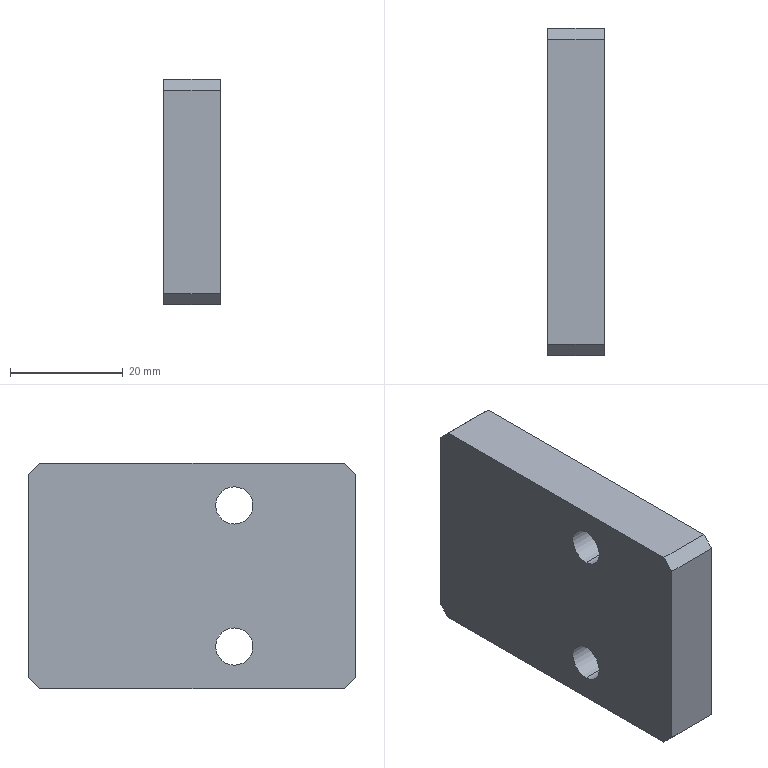Component | SolidWorks | NewDieSet-1_MoldSlotBaffle-7 | 1 solid | 14 faces | box 10 x 58 x 40 mm | volume 22436 mm3 | plane 10 | cylinder 4 | commonest cylinder face diameters 6.6 x4
build123d program:
from build123d import *

# Parameters (mm, degrees)
SKETCH1_W                = 58
SKETCH1_H                = 40
BOSS_EXTRUDE1_DEPTH      = 10
CHAMFER1_SIZE            = 2
M6_CLEARANCE_HOLE1_D     = 6.6
M6_CLEARANCE_HOLE1_DEPTH = 25.2
M6_CLEARANCE_HOLE1_TIP   = 1.983


with BuildPart() as part:
    # Sketch1 → Boss-Extrude1 (new body)
    with BuildSketch(Plane(origin=(0, 0, 0), x_dir=(1, 0, 0), z_dir=(0, 1, 0))):
        with Locations((29, 20)):
            Rectangle(SKETCH1_W, SKETCH1_H)
    extrude(amount=BOSS_EXTRUDE1_DEPTH)

    # Chamfer1
    chamfer1_edges = [part.edges().sort_by_distance(p)[0] for p in [
        (0, 5, -40),
        (58, 5, -40),
        (58, 5, 0),
        (0, 5, 0),
    ]]
    chamfer(chamfer1_edges, length=CHAMFER1_SIZE)

    # M6 Clearance Hole1
    with Locations(Plane(origin=(0, 10, 0), x_dir=(1, 0, 0), z_dir=(0, 1, 0))):
        with Locations((36.5, 7.5), (36.5, 32.5)):
            Hole(M6_CLEARANCE_HOLE1_D / 2, depth=M6_CLEARANCE_HOLE1_DEPTH)
            with Locations((0, 0, -(M6_CLEARANCE_HOLE1_DEPTH + M6_CLEARANCE_HOLE1_TIP / 2))):  # 118° drill point
                Cone(0, M6_CLEARANCE_HOLE1_D / 2, M6_CLEARANCE_HOLE1_TIP, mode=Mode.SUBTRACT)


solid = part.part

# Placed as in the assembly
solid = solid.moved(Location((143.254, 22.427, 215.5), (0, 0, -90)))
STEP:
#1=COLOUR_RGB('',0.7922,0.8196,0.9333);
#2=FILL_AREA_STYLE_COLOUR('',#1);
#3=FILL_AREA_STYLE('',(#2));
#4=SURFACE_STYLE_FILL_AREA(#3);
#5=SURFACE_SIDE_STYLE('',(#4));
#6=SURFACE_STYLE_USAGE(.BOTH.,#5);
#7=PRESENTATION_STYLE_ASSIGNMENT((#6));
#8=CARTESIAN_POINT('',(5.64,-0.5541,8.319));
#9=VERTEX_POINT('',#8);
#10=CARTESIAN_POINT('',(5.64,-0.5541,8.059));
#11=VERTEX_POINT('',#10);
#12=CARTESIAN_POINT('',(5.64,-0.5541,8.189));
#13=DIRECTION('',(-1.,0.,-0.));
#14=DIRECTION('',(0.,0.,-1.));
#15=AXIS2_PLACEMENT_3D('',#12,#13,#14);
#16=CIRCLE('',#15,0.1299);
#17=EDGE_CURVE('',#9,#11,#16,.T.);
#18=ORIENTED_EDGE('',*,*,#17,.T.);
#19=CARTESIAN_POINT('',(6.034,-0.5541,8.059));
#20=VERTEX_POINT('',#19);
#21=CARTESIAN_POINT('',(6.034,-0.5541,8.059));
#22=DIRECTION('',(1.,-0.,0.));
#23=VECTOR('',#22,39.37);
#24=LINE('',#21,#23);
#25=EDGE_CURVE('',#11,#20,#24,.T.);
#26=ORIENTED_EDGE('',*,*,#25,.T.);
#27=CARTESIAN_POINT('',(6.034,-0.5541,8.319));
#28=VERTEX_POINT('',#27);
#29=CARTESIAN_POINT('',(6.034,-0.5541,8.189));
#30=DIRECTION('',(1.,-0.,0.));
#31=DIRECTION('',(0.,0.,1.));
#32=AXIS2_PLACEMENT_3D('',#29,#30,#31);
#33=CIRCLE('',#32,0.1299);
#34=EDGE_CURVE('',#20,#28,#33,.T.);
#35=ORIENTED_EDGE('',*,*,#34,.T.);
#36=CARTESIAN_POINT('',(6.034,-0.5541,8.319));
#37=DIRECTION('',(1.,-0.,0.));
#38=VECTOR('',#37,39.37);
#39=LINE('',#36,#38);
#40=EDGE_CURVE('',#9,#28,#39,.T.);
#41=ORIENTED_EDGE('',*,*,#40,.F.);
#42=EDGE_LOOP('',(#18,#26,#35,#41));
#43=FACE_OUTER_BOUND('',#42,.T.);
#44=CARTESIAN_POINT('',(6.034,-0.5541,8.189));
#45=DIRECTION('',(1.,-0.,0.));
#46=DIRECTION('',(0.,0.,1.));
#47=AXIS2_PLACEMENT_3D('',#44,#45,#46);
#48=CYLINDRICAL_SURFACE('',#47,0.1299);
#49=ADVANCED_FACE('',(#43),#48,.F.);
#50=CARTESIAN_POINT('',(5.64,-0.5541,7.335));
#51=VERTEX_POINT('',#50);
#52=CARTESIAN_POINT('',(5.64,-0.5541,7.075));
#53=VERTEX_POINT('',#52);
#54=CARTESIAN_POINT('',(5.64,-0.5541,7.205));
#55=DIRECTION('',(-1.,0.,-0.));
#56=DIRECTION('',(0.,0.,-1.));
#57=AXIS2_PLACEMENT_3D('',#54,#55,#56);
#58=CIRCLE('',#57,0.1299);
#59=EDGE_CURVE('',#51,#53,#58,.T.);
#60=ORIENTED_EDGE('',*,*,#59,.T.);
#61=CARTESIAN_POINT('',(6.034,-0.5541,7.075));
#62=VERTEX_POINT('',#61);
#63=CARTESIAN_POINT('',(6.034,-0.5541,7.075));
#64=DIRECTION('',(1.,-0.,0.));
#65=VECTOR('',#64,39.37);
#66=LINE('',#63,#65);
#67=EDGE_CURVE('',#53,#62,#66,.T.);
#68=ORIENTED_EDGE('',*,*,#67,.T.);
#69=CARTESIAN_POINT('',(6.034,-0.5541,7.335));
#70=VERTEX_POINT('',#69);
#71=CARTESIAN_POINT('',(6.034,-0.5541,7.205));
#72=DIRECTION('',(1.,-0.,0.));
#73=DIRECTION('',(0.,0.,1.));
#74=AXIS2_PLACEMENT_3D('',#71,#72,#73);
#75=CIRCLE('',#74,0.1299);
#76=EDGE_CURVE('',#62,#70,#75,.T.);
#77=ORIENTED_EDGE('',*,*,#76,.T.);
#78=CARTESIAN_POINT('',(6.034,-0.5541,7.335));
#79=DIRECTION('',(1.,-0.,0.));
#80=VECTOR('',#79,39.37);
#81=LINE('',#78,#80);
#82=EDGE_CURVE('',#51,#70,#81,.T.);
#83=ORIENTED_EDGE('',*,*,#82,.F.);
#84=EDGE_LOOP('',(#60,#68,#77,#83));
#85=FACE_OUTER_BOUND('',#84,.T.);
#86=CARTESIAN_POINT('',(6.034,-0.5541,7.205));
#87=DIRECTION('',(1.,-0.,0.));
#88=DIRECTION('',(0.,0.,1.));
#89=AXIS2_PLACEMENT_3D('',#86,#87,#88);
#90=CYLINDRICAL_SURFACE('',#89,0.1299);
#91=ADVANCED_FACE('',(#85),#90,.F.);
#92=CARTESIAN_POINT('',(5.64,0.883,6.988));
#93=VERTEX_POINT('',#92);
#94=CARTESIAN_POINT('',(5.64,0.883,8.406));
#95=VERTEX_POINT('',#94);
#96=CARTESIAN_POINT('',(5.64,0.883,8.484));
#97=DIRECTION('',(-0.,0.,1.));
#98=VECTOR('',#97,39.37);
#99=LINE('',#96,#98);
#100=EDGE_CURVE('',#93,#95,#99,.T.);
#101=ORIENTED_EDGE('',*,*,#100,.T.);
#102=CARTESIAN_POINT('',(6.034,0.883,8.406));
#103=VERTEX_POINT('',#102);
#104=CARTESIAN_POINT('',(6.034,0.883,8.406));
#105=DIRECTION('',(1.,-0.,0.));
#106=VECTOR('',#105,39.37);
#107=LINE('',#104,#106);
#108=EDGE_CURVE('',#95,#103,#107,.T.);
#109=ORIENTED_EDGE('',*,*,#108,.T.);
#110=CARTESIAN_POINT('',(6.034,0.883,6.988));
#111=VERTEX_POINT('',#110);
#112=CARTESIAN_POINT('',(6.034,0.883,8.484));
#113=DIRECTION('',(-0.,0.,1.));
#114=VECTOR('',#113,39.37);
#115=LINE('',#112,#114);
#116=EDGE_CURVE('',#111,#103,#115,.T.);
#117=ORIENTED_EDGE('',*,*,#116,.F.);
#118=CARTESIAN_POINT('',(6.034,0.883,6.988));
#119=DIRECTION('',(-1.,0.,-0.));
#120=VECTOR('',#119,39.37);
#121=LINE('',#118,#120);
#122=EDGE_CURVE('',#111,#93,#121,.T.);
#123=ORIENTED_EDGE('',*,*,#122,.T.);
#124=EDGE_LOOP('',(#101,#109,#117,#123));
#125=FACE_OUTER_BOUND('',#124,.T.);
#126=CARTESIAN_POINT('',(6.034,0.883,8.484));
#127=DIRECTION('',(-0.,-1.,0.));
#128=DIRECTION('',(0.,-0.,-1.));
#129=AXIS2_PLACEMENT_3D('',#126,#127,#128);
#130=PLANE('',#129);
#131=ADVANCED_FACE('',(#125),#130,.F.);
#132=CARTESIAN_POINT('',(6.034,0.8042,8.484));
#133=VERTEX_POINT('',#132);
#134=CARTESIAN_POINT('',(6.034,-1.322,8.484));
#135=VERTEX_POINT('',#134);
#136=CARTESIAN_POINT('',(6.034,0.883,8.484));
#137=DIRECTION('',(-0.,-1.,0.));
#138=VECTOR('',#137,39.37);
#139=LINE('',#136,#138);
#140=EDGE_CURVE('',#133,#135,#139,.T.);
#141=ORIENTED_EDGE('',*,*,#140,.F.);
#142=CARTESIAN_POINT('',(5.64,0.8042,8.484));
#143=VERTEX_POINT('',#142);
#144=CARTESIAN_POINT('',(6.034,0.8042,8.484));
#145=DIRECTION('',(-1.,0.,-0.));
#146=VECTOR('',#145,39.37);
#147=LINE('',#144,#146);
#148=EDGE_CURVE('',#133,#143,#147,.T.);
#149=ORIENTED_EDGE('',*,*,#148,.T.);
#150=CARTESIAN_POINT('',(5.64,-1.322,8.484));
#151=VERTEX_POINT('',#150);
#152=CARTESIAN_POINT('',(5.64,0.883,8.484));
#153=DIRECTION('',(-0.,-1.,0.));
#154=VECTOR('',#153,39.37);
#155=LINE('',#152,#154);
#156=EDGE_CURVE('',#143,#151,#155,.T.);
#157=ORIENTED_EDGE('',*,*,#156,.T.);
#158=CARTESIAN_POINT('',(6.034,-1.322,8.484));
#159=DIRECTION('',(1.,-0.,0.));
#160=VECTOR('',#159,39.37);
#161=LINE('',#158,#160);
#162=EDGE_CURVE('',#151,#135,#161,.T.);
#163=ORIENTED_EDGE('',*,*,#162,.T.);
#164=EDGE_LOOP('',(#141,#149,#157,#163));
#165=FACE_OUTER_BOUND('',#164,.T.);
#166=CARTESIAN_POINT('',(6.034,0.883,8.484));
#167=DIRECTION('',(0.,-0.,-1.));
#168=DIRECTION('',(0.,1.,-0.));
#169=AXIS2_PLACEMENT_3D('',#166,#167,#168);
#170=PLANE('',#169);
#171=ADVANCED_FACE('',(#165),#170,.F.);
#172=CARTESIAN_POINT('',(6.034,-1.401,8.406));
#173=VERTEX_POINT('',#172);
#174=CARTESIAN_POINT('',(6.034,-1.401,6.988));
#175=VERTEX_POINT('',#174);
#176=CARTESIAN_POINT('',(6.034,-1.401,8.484));
#177=DIRECTION('',(0.,-0.,-1.));
#178=VECTOR('',#177,39.37);
#179=LINE('',#176,#178);
#180=EDGE_CURVE('',#173,#175,#179,.T.);
#181=ORIENTED_EDGE('',*,*,#180,.F.);
#182=CARTESIAN_POINT('',(5.64,-1.401,8.406));
#183=VERTEX_POINT('',#182);
#184=CARTESIAN_POINT('',(6.034,-1.401,8.406));
#185=DIRECTION('',(-1.,0.,-0.));
#186=VECTOR('',#185,39.37);
#187=LINE('',#184,#186);
#188=EDGE_CURVE('',#173,#183,#187,.T.);
#189=ORIENTED_EDGE('',*,*,#188,.T.);
#190=CARTESIAN_POINT('',(5.64,-1.401,6.988));
#191=VERTEX_POINT('',#190);
#192=CARTESIAN_POINT('',(5.64,-1.401,8.484));
#193=DIRECTION('',(0.,-0.,-1.));
#194=VECTOR('',#193,39.37);
#195=LINE('',#192,#194);
#196=EDGE_CURVE('',#183,#191,#195,.T.);
#197=ORIENTED_EDGE('',*,*,#196,.T.);
#198=CARTESIAN_POINT('',(6.034,-1.401,6.988));
#199=DIRECTION('',(1.,-0.,0.));
#200=VECTOR('',#199,39.37);
#201=LINE('',#198,#200);
#202=EDGE_CURVE('',#191,#175,#201,.T.);
#203=ORIENTED_EDGE('',*,*,#202,.T.);
#204=EDGE_LOOP('',(#181,#189,#197,#203));
#205=FACE_OUTER_BOUND('',#204,.T.);
#206=CARTESIAN_POINT('',(6.034,-1.401,8.484));
#207=DIRECTION('',(0.,1.,-0.));
#208=DIRECTION('',(-0.,0.,1.));
#209=AXIS2_PLACEMENT_3D('',#206,#207,#208);
#210=PLANE('',#209);
#211=ADVANCED_FACE('',(#205),#210,.F.);
#212=CARTESIAN_POINT('',(6.034,-1.322,6.909));
#213=VERTEX_POINT('',#212);
#214=CARTESIAN_POINT('',(6.034,0.8042,6.909));
#215=VERTEX_POINT('',#214);
#216=CARTESIAN_POINT('',(6.034,0.883,6.909));
#217=DIRECTION('',(0.,1.,-0.));
#218=VECTOR('',#217,39.37);
#219=LINE('',#216,#218);
#220=EDGE_CURVE('',#213,#215,#219,.T.);
#221=ORIENTED_EDGE('',*,*,#220,.F.);
#222=CARTESIAN_POINT('',(5.64,-1.322,6.909));
#223=VERTEX_POINT('',#222);
#224=CARTESIAN_POINT('',(6.034,-1.322,6.909));
#225=DIRECTION('',(-1.,0.,-0.));
#226=VECTOR('',#225,39.37);
#227=LINE('',#224,#226);
#228=EDGE_CURVE('',#213,#223,#227,.T.);
#229=ORIENTED_EDGE('',*,*,#228,.T.);
#230=CARTESIAN_POINT('',(5.64,0.8042,6.909));
#231=VERTEX_POINT('',#230);
#232=CARTESIAN_POINT('',(5.64,0.883,6.909));
#233=DIRECTION('',(0.,1.,-0.));
#234=VECTOR('',#233,39.37);
#235=LINE('',#232,#234);
#236=EDGE_CURVE('',#223,#231,#235,.T.);
#237=ORIENTED_EDGE('',*,*,#236,.T.);
#238=CARTESIAN_POINT('',(6.034,0.8042,6.909));
#239=DIRECTION('',(1.,-0.,0.));
#240=VECTOR('',#239,39.37);
#241=LINE('',#238,#240);
#242=EDGE_CURVE('',#231,#215,#241,.T.);
#243=ORIENTED_EDGE('',*,*,#242,.T.);
#244=EDGE_LOOP('',(#221,#229,#237,#243));
#245=FACE_OUTER_BOUND('',#244,.T.);
#246=CARTESIAN_POINT('',(6.034,0.883,6.909));
#247=DIRECTION('',(-0.,0.,1.));
#248=DIRECTION('',(-0.,-1.,0.));
#249=AXIS2_PLACEMENT_3D('',#246,#247,#248);
#250=PLANE('',#249);
#251=ADVANCED_FACE('',(#245),#250,.F.);
#252=CARTESIAN_POINT('',(6.034,-0.5541,8.189));
#253=DIRECTION('',(1.,-0.,0.));
#254=DIRECTION('',(0.,0.,1.));
#255=AXIS2_PLACEMENT_3D('',#252,#253,#254);
#256=CIRCLE('',#255,0.1299);
#257=EDGE_CURVE('',#28,#20,#256,.T.);
#258=ORIENTED_EDGE('',*,*,#257,.F.);
#259=ORIENTED_EDGE('',*,*,#34,.F.);
#260=EDGE_LOOP('',(#258,#259));
#261=FACE_BOUND('',#260,.T.);
#262=CARTESIAN_POINT('',(6.034,-0.5541,7.205));
#263=DIRECTION('',(1.,-0.,0.));
#264=DIRECTION('',(0.,0.,1.));
#265=AXIS2_PLACEMENT_3D('',#262,#263,#264);
#266=CIRCLE('',#265,0.1299);
#267=EDGE_CURVE('',#70,#62,#266,.T.);
#268=ORIENTED_EDGE('',*,*,#267,.F.);
#269=ORIENTED_EDGE('',*,*,#76,.F.);
#270=EDGE_LOOP('',(#268,#269));
#271=FACE_BOUND('',#270,.T.);
#272=ORIENTED_EDGE('',*,*,#116,.T.);
#273=CARTESIAN_POINT('',(6.034,0.8042,8.484));
#274=DIRECTION('',(-0.,-0.7071,0.7071));
#275=VECTOR('',#274,39.37);
#276=LINE('',#273,#275);
#277=EDGE_CURVE('',#103,#133,#276,.T.);
#278=ORIENTED_EDGE('',*,*,#277,.T.);
#279=ORIENTED_EDGE('',*,*,#140,.T.);
#280=CARTESIAN_POINT('',(6.034,-1.401,8.406));
#281=DIRECTION('',(0.,-0.7071,-0.7071));
#282=VECTOR('',#281,39.37);
#283=LINE('',#280,#282);
#284=EDGE_CURVE('',#135,#173,#283,.T.);
#285=ORIENTED_EDGE('',*,*,#284,.T.);
#286=ORIENTED_EDGE('',*,*,#180,.T.);
#287=CARTESIAN_POINT('',(6.034,-1.322,6.909));
#288=DIRECTION('',(0.,0.7071,-0.7071));
#289=VECTOR('',#288,39.37);
#290=LINE('',#287,#289);
#291=EDGE_CURVE('',#175,#213,#290,.T.);
#292=ORIENTED_EDGE('',*,*,#291,.T.);
#293=ORIENTED_EDGE('',*,*,#220,.T.);
#294=CARTESIAN_POINT('',(6.034,0.883,6.988));
#295=DIRECTION('',(-0.,0.7071,0.7071));
#296=VECTOR('',#295,39.37);
#297=LINE('',#294,#296);
#298=EDGE_CURVE('',#215,#111,#297,.T.);
#299=ORIENTED_EDGE('',*,*,#298,.T.);
#300=EDGE_LOOP('',(#272,#278,#279,#285,#286,#292,#293,#299));
#301=FACE_OUTER_BOUND('',#300,.T.);
#302=CARTESIAN_POINT('',(6.034,0.883,8.484));
#303=DIRECTION('',(-1.,0.,-0.));
#304=DIRECTION('',(0.,-0.,-1.));
#305=AXIS2_PLACEMENT_3D('',#302,#303,#304);
#306=PLANE('',#305);
#307=ADVANCED_FACE('',(#261,#271,#301),#306,.F.);
#308=ORIENTED_EDGE('',*,*,#17,.F.);
#309=CARTESIAN_POINT('',(5.64,-0.5541,8.189));
#310=DIRECTION('',(-1.,0.,-0.));
#311=DIRECTION('',(0.,0.,-1.));
#312=AXIS2_PLACEMENT_3D('',#309,#310,#311);
#313=CIRCLE('',#312,0.1299);
#314=EDGE_CURVE('',#11,#9,#313,.T.);
#315=ORIENTED_EDGE('',*,*,#314,.F.);
#316=EDGE_LOOP('',(#308,#315));
#317=FACE_BOUND('',#316,.T.);
#318=ORIENTED_EDGE('',*,*,#59,.F.);
#319=CARTESIAN_POINT('',(5.64,-0.5541,7.205));
#320=DIRECTION('',(-1.,0.,-0.));
#321=DIRECTION('',(0.,0.,-1.));
#322=AXIS2_PLACEMENT_3D('',#319,#320,#321);
#323=CIRCLE('',#322,0.1299);
#324=EDGE_CURVE('',#53,#51,#323,.T.);
#325=ORIENTED_EDGE('',*,*,#324,.F.);
#326=EDGE_LOOP('',(#318,#325));
#327=FACE_BOUND('',#326,.T.);
#328=ORIENTED_EDGE('',*,*,#156,.F.);
#329=CARTESIAN_POINT('',(5.64,0.8436,8.445));
#330=DIRECTION('',(0.,0.7071,-0.7071));
#331=VECTOR('',#330,39.37);
#332=LINE('',#329,#331);
#333=EDGE_CURVE('',#143,#95,#332,.T.);
#334=ORIENTED_EDGE('',*,*,#333,.T.);
#335=ORIENTED_EDGE('',*,*,#100,.F.);
#336=CARTESIAN_POINT('',(5.64,1.631,7.736));
#337=DIRECTION('',(0.,-0.7071,-0.7071));
#338=VECTOR('',#337,39.37);
#339=LINE('',#336,#338);
#340=EDGE_CURVE('',#93,#231,#339,.T.);
#341=ORIENTED_EDGE('',*,*,#340,.T.);
#342=ORIENTED_EDGE('',*,*,#236,.F.);
#343=CARTESIAN_POINT('',(5.64,-1.007,6.594));
#344=DIRECTION('',(-0.,-0.7071,0.7071));
#345=VECTOR('',#344,39.37);
#346=LINE('',#343,#345);
#347=EDGE_CURVE('',#223,#191,#346,.T.);
#348=ORIENTED_EDGE('',*,*,#347,.T.);
#349=ORIENTED_EDGE('',*,*,#196,.F.);
#350=CARTESIAN_POINT('',(5.64,-0.2194,9.587));
#351=DIRECTION('',(-0.,0.7071,0.7071));
#352=VECTOR('',#351,39.37);
#353=LINE('',#350,#352);
#354=EDGE_CURVE('',#183,#151,#353,.T.);
#355=ORIENTED_EDGE('',*,*,#354,.T.);
#356=EDGE_LOOP('',(#328,#334,#335,#341,#342,#348,#349,#355));
#357=FACE_OUTER_BOUND('',#356,.T.);
#358=CARTESIAN_POINT('',(5.64,0.883,8.484));
#359=DIRECTION('',(-1.,0.,-0.));
#360=DIRECTION('',(0.,-0.,-1.));
#361=AXIS2_PLACEMENT_3D('',#358,#359,#360);
#362=PLANE('',#361);
#363=ADVANCED_FACE('',(#317,#327,#357),#362,.T.);
#364=ORIENTED_EDGE('',*,*,#277,.F.);
#365=ORIENTED_EDGE('',*,*,#108,.F.);
#366=ORIENTED_EDGE('',*,*,#333,.F.);
#367=ORIENTED_EDGE('',*,*,#148,.F.);
#368=EDGE_LOOP('',(#364,#365,#366,#367));
#369=FACE_OUTER_BOUND('',#368,.T.);
#370=CARTESIAN_POINT('',(6.034,0.8042,8.484));
#371=DIRECTION('',(0.,-0.7071,-0.7071));
#372=DIRECTION('',(-1.,0.,-0.));
#373=AXIS2_PLACEMENT_3D('',#370,#371,#372);
#374=PLANE('',#373);
#375=ADVANCED_FACE('',(#369),#374,.F.);
#376=ORIENTED_EDGE('',*,*,#284,.F.);
#377=ORIENTED_EDGE('',*,*,#162,.F.);
#378=ORIENTED_EDGE('',*,*,#354,.F.);
#379=ORIENTED_EDGE('',*,*,#188,.F.);
#380=EDGE_LOOP('',(#376,#377,#378,#379));
#381=FACE_OUTER_BOUND('',#380,.T.);
#382=CARTESIAN_POINT('',(6.034,-1.401,8.406));
#383=DIRECTION('',(0.,0.7071,-0.7071));
#384=DIRECTION('',(-1.,0.,-0.));
#385=AXIS2_PLACEMENT_3D('',#382,#383,#384);
#386=PLANE('',#385);
#387=ADVANCED_FACE('',(#381),#386,.F.);
#388=ORIENTED_EDGE('',*,*,#291,.F.);
#389=ORIENTED_EDGE('',*,*,#202,.F.);
#390=ORIENTED_EDGE('',*,*,#347,.F.);
#391=ORIENTED_EDGE('',*,*,#228,.F.);
#392=EDGE_LOOP('',(#388,#389,#390,#391));
#393=FACE_OUTER_BOUND('',#392,.T.);
#394=CARTESIAN_POINT('',(6.034,-1.322,6.909));
#395=DIRECTION('',(-0.,0.7071,0.7071));
#396=DIRECTION('',(-1.,0.,-0.));
#397=AXIS2_PLACEMENT_3D('',#394,#395,#396);
#398=PLANE('',#397);
#399=ADVANCED_FACE('',(#393),#398,.F.);
#400=ORIENTED_EDGE('',*,*,#298,.F.);
#401=ORIENTED_EDGE('',*,*,#242,.F.);
#402=ORIENTED_EDGE('',*,*,#340,.F.);
#403=ORIENTED_EDGE('',*,*,#122,.F.);
#404=EDGE_LOOP('',(#400,#401,#402,#403));
#405=FACE_OUTER_BOUND('',#404,.T.);
#406=CARTESIAN_POINT('',(6.034,0.883,6.988));
#407=DIRECTION('',(-0.,-0.7071,0.7071));
#408=DIRECTION('',(-1.,0.,-0.));
#409=AXIS2_PLACEMENT_3D('',#406,#407,#408);
#410=PLANE('',#409);
#411=ADVANCED_FACE('',(#405),#410,.F.);
#412=ORIENTED_EDGE('',*,*,#67,.F.);
#413=ORIENTED_EDGE('',*,*,#324,.T.);
#414=ORIENTED_EDGE('',*,*,#82,.T.);
#415=ORIENTED_EDGE('',*,*,#267,.T.);
#416=EDGE_LOOP('',(#412,#413,#414,#415));
#417=FACE_OUTER_BOUND('',#416,.T.);
#418=CARTESIAN_POINT('',(6.034,-0.5541,7.205));
#419=DIRECTION('',(1.,-0.,0.));
#420=DIRECTION('',(0.,0.,1.));
#421=AXIS2_PLACEMENT_3D('',#418,#419,#420);
#422=CYLINDRICAL_SURFACE('',#421,0.1299);
#423=ADVANCED_FACE('',(#417),#422,.F.);
#424=ORIENTED_EDGE('',*,*,#25,.F.);
#425=ORIENTED_EDGE('',*,*,#314,.T.);
#426=ORIENTED_EDGE('',*,*,#40,.T.);
#427=ORIENTED_EDGE('',*,*,#257,.T.);
#428=EDGE_LOOP('',(#424,#425,#426,#427));
#429=FACE_OUTER_BOUND('',#428,.T.);
#430=CARTESIAN_POINT('',(6.034,-0.5541,8.189));
#431=DIRECTION('',(1.,-0.,0.));
#432=DIRECTION('',(0.,0.,1.));
#433=AXIS2_PLACEMENT_3D('',#430,#431,#432);
#434=CYLINDRICAL_SURFACE('',#433,0.1299);
#435=ADVANCED_FACE('',(#429),#434,.F.);
#436=CLOSED_SHELL('',(#49,#91,#131,#171,#211,#251,#307,#363,#375,#387,#399,#411,#423,#435));
#437=MANIFOLD_SOLID_BREP('',#436);
#438=STYLED_ITEM('',(#7),#437);
#439=(LENGTH_UNIT()NAMED_UNIT(*)SI_UNIT($,.METRE.));
#440=LENGTH_MEASURE_WITH_UNIT(LENGTH_MEASURE(0.0254),#439);
#441=DIMENSIONAL_EXPONENTS(1.,0.,0.,0.,0.,0.,0.);
#442=(CONVERSION_BASED_UNIT('',#440)LENGTH_UNIT()NAMED_UNIT(#441));
#443=UNCERTAINTY_MEASURE_WITH_UNIT(LENGTH_MEASURE(0.00001),#442,'','');
#444=(NAMED_UNIT(*)PLANE_ANGLE_UNIT()SI_UNIT($,.RADIAN.));
#445=(NAMED_UNIT(*)SI_UNIT($,.STERADIAN.)SOLID_ANGLE_UNIT());
#446=(GEOMETRIC_REPRESENTATION_CONTEXT(3)GLOBAL_UNCERTAINTY_ASSIGNED_CONTEXT((#443))GLOBAL_UNIT_ASSIGNED_CONTEXT((#442,#444,#445))REPRESENTATION_CONTEXT('',''));
#447=MECHANICAL_DESIGN_GEOMETRIC_PRESENTATION_REPRESENTATION('',(#438),#446);
#448=PRESENTATION_LAYER_ASSIGNMENT('','',(#438));
#449=CARTESIAN_POINT('',(0.,0.,0.));
#450=DIRECTION('',(0.,0.,1.));
#451=DIRECTION('',(1.,0.,0.));
#452=AXIS2_PLACEMENT_3D('',#449,#450,#451);
#453=(LENGTH_UNIT()NAMED_UNIT(*)SI_UNIT($,.METRE.));
#454=LENGTH_MEASURE_WITH_UNIT(LENGTH_MEASURE(0.0254),#453);
#455=DIMENSIONAL_EXPONENTS(1.,0.,0.,0.,0.,0.,0.);
#456=(CONVERSION_BASED_UNIT('',#454)LENGTH_UNIT()NAMED_UNIT(#455));
#457=UNCERTAINTY_MEASURE_WITH_UNIT(LENGTH_MEASURE(0.00001),#456,'','');
#458=(NAMED_UNIT(*)PLANE_ANGLE_UNIT()SI_UNIT($,.RADIAN.));
#459=(NAMED_UNIT(*)SI_UNIT($,.STERADIAN.)SOLID_ANGLE_UNIT());
#460=(GEOMETRIC_REPRESENTATION_CONTEXT(3)GLOBAL_UNCERTAINTY_ASSIGNED_CONTEXT((#457))GLOBAL_UNIT_ASSIGNED_CONTEXT((#456,#458,#459))REPRESENTATION_CONTEXT('',''));
#461=ADVANCED_BREP_SHAPE_REPRESENTATION('',(#437,#452),#460);